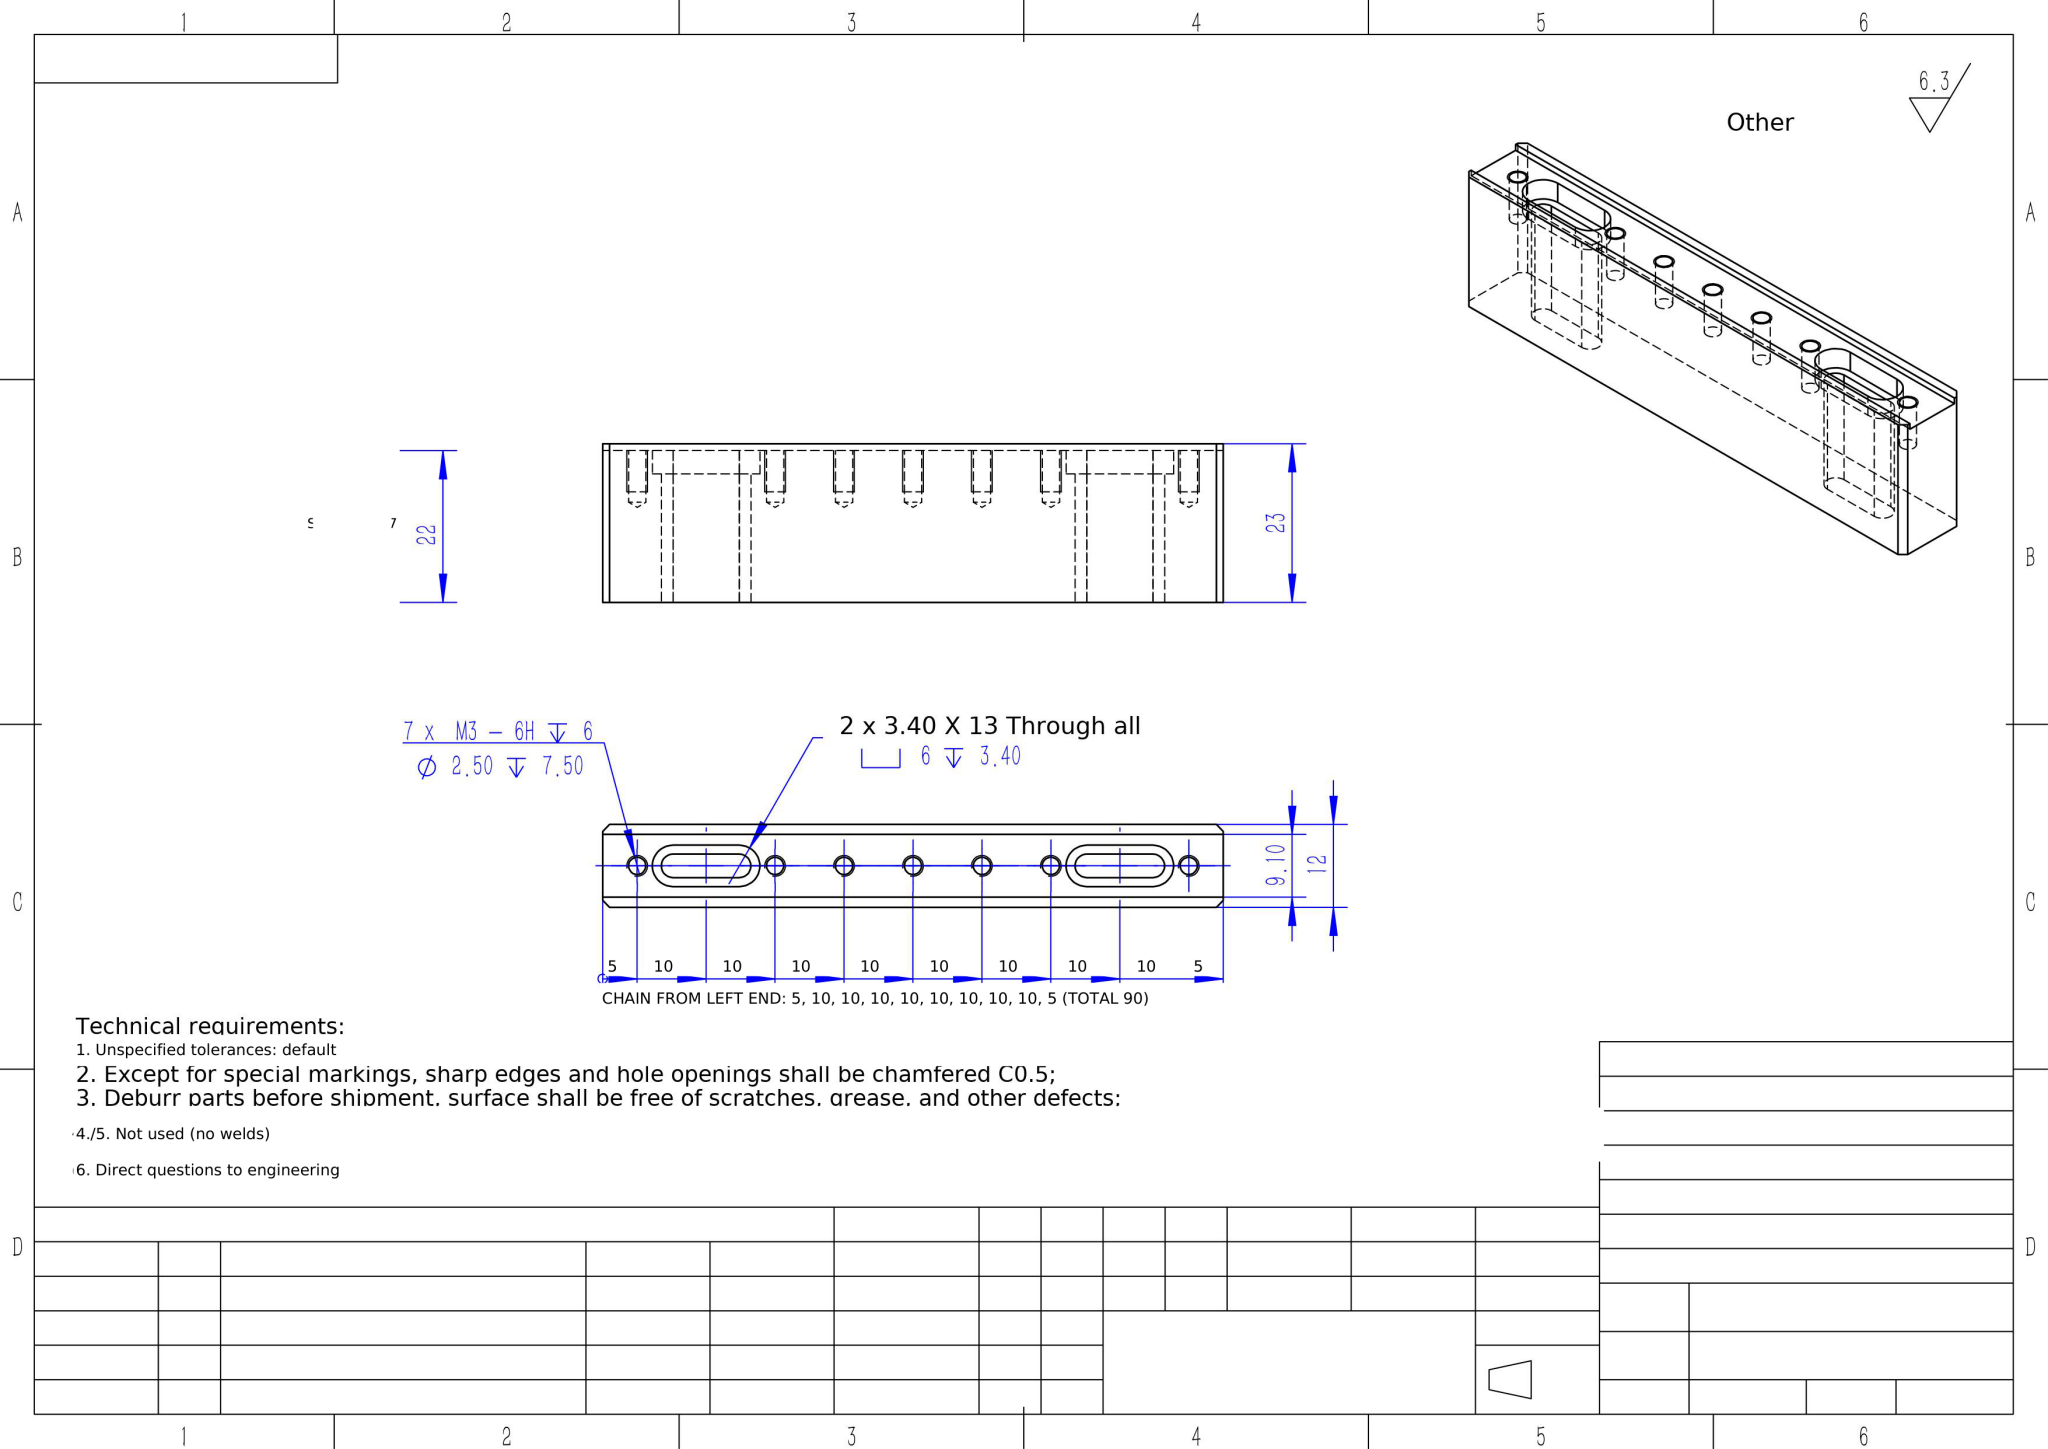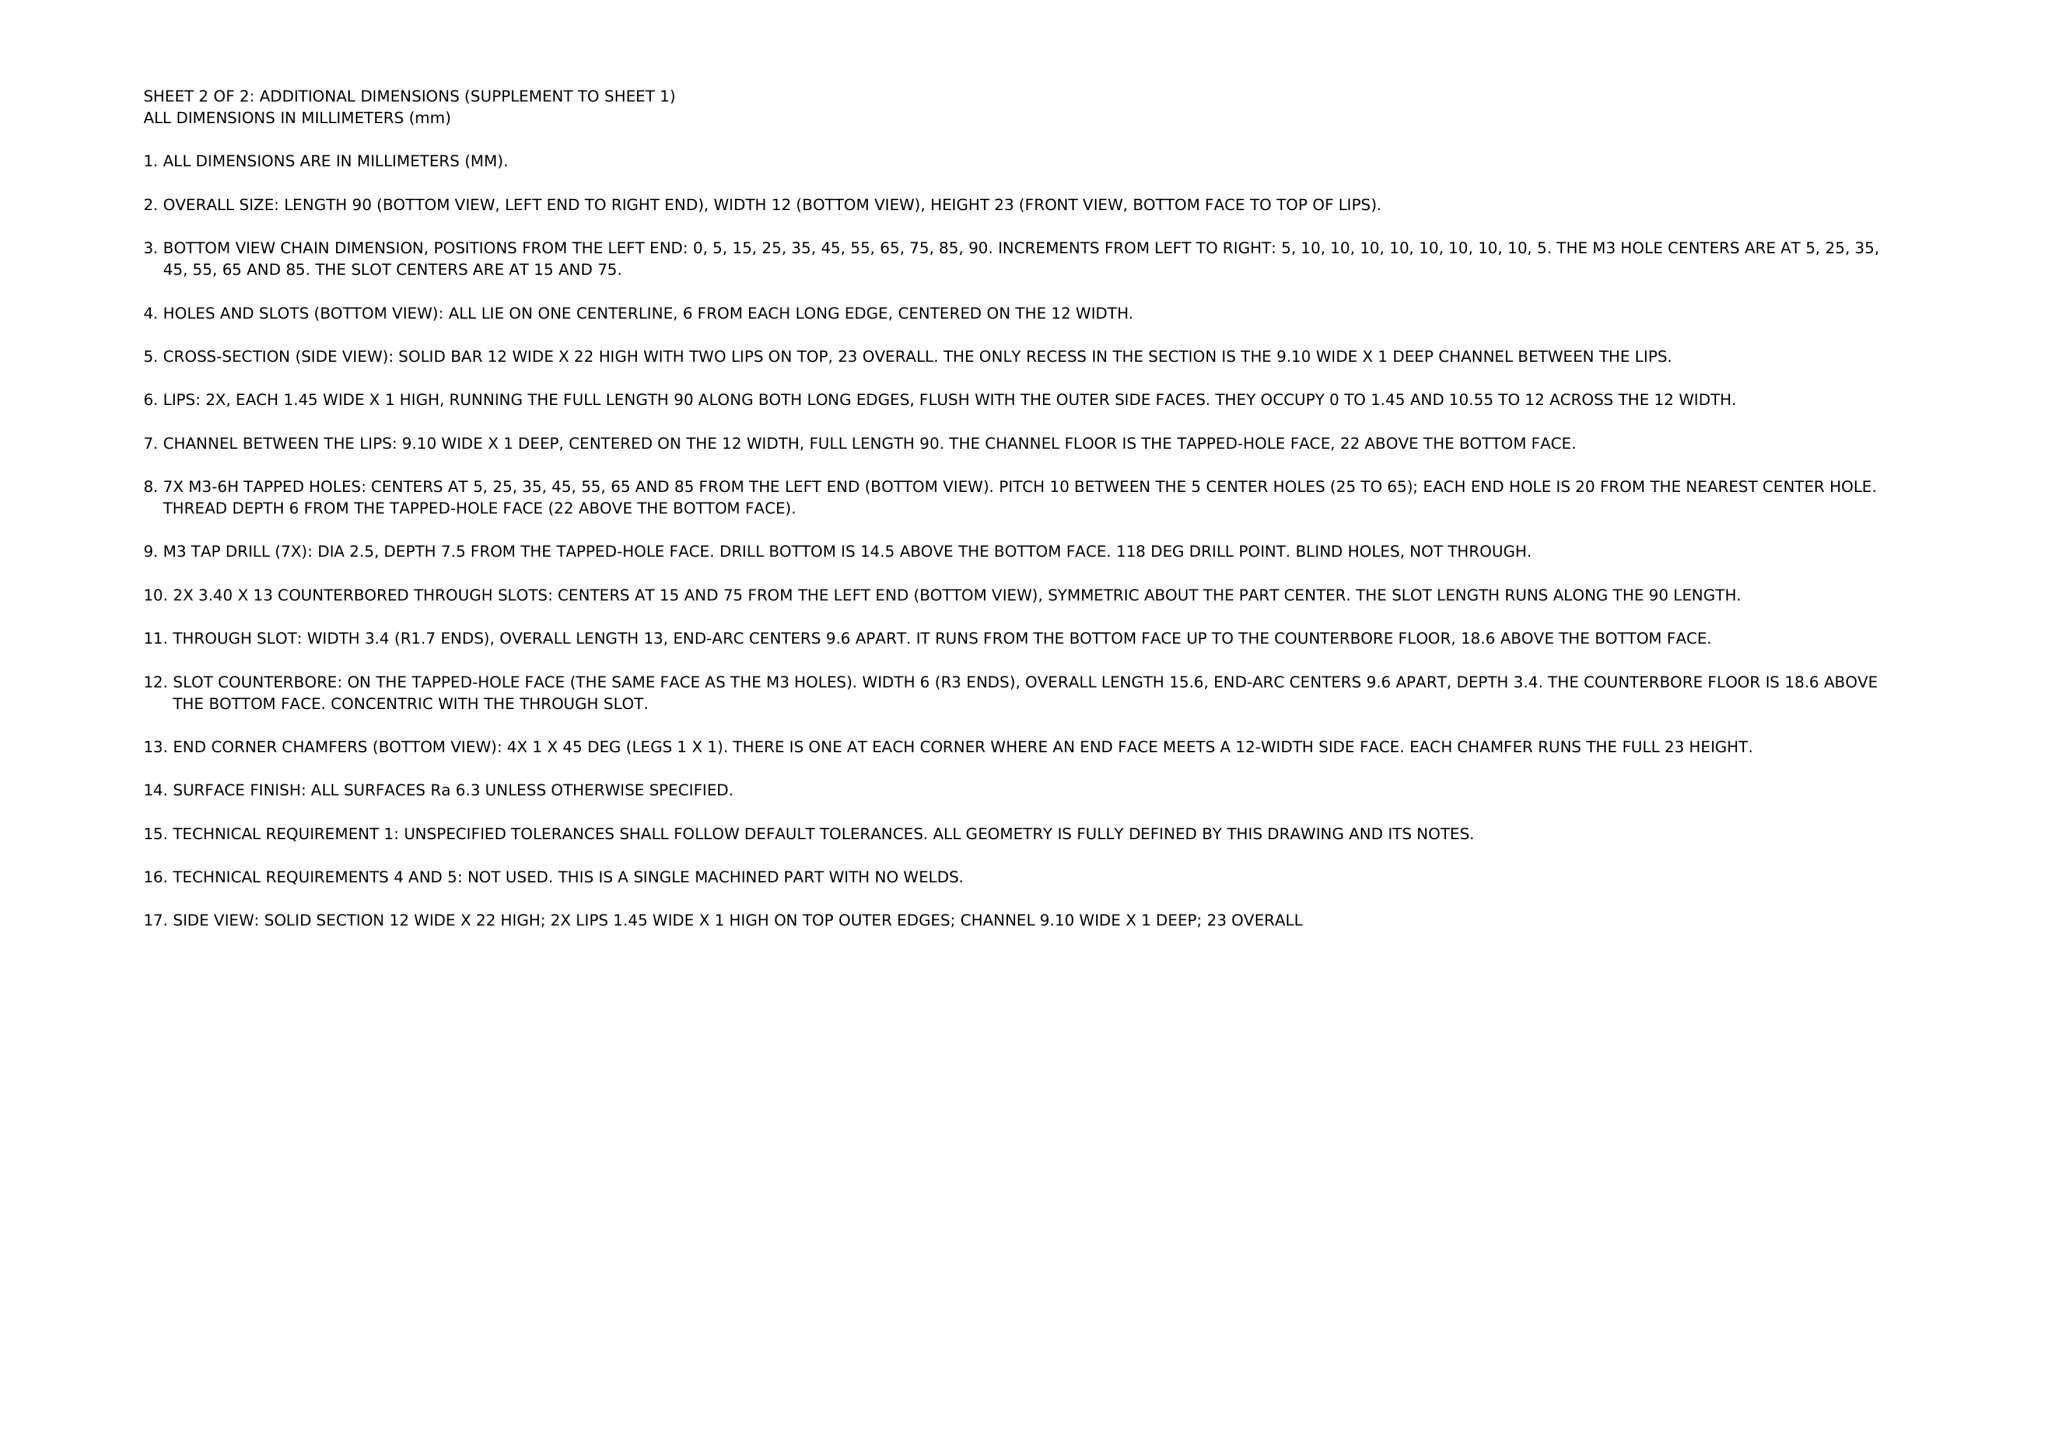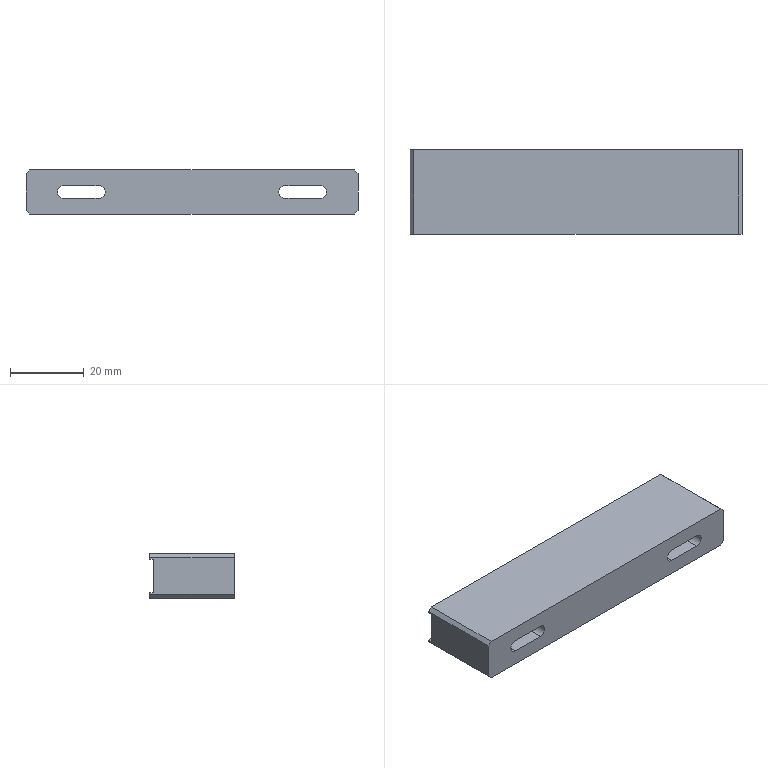Part | NX | mm | 1 solid | 60 faces | box 90 x 23 x 12 mm | volume 21573 mm3 | plane 24 | cylinder 22 | cone 14 | commonest cylinder face diameters 2.5 x14 3.4 x4 6 x4